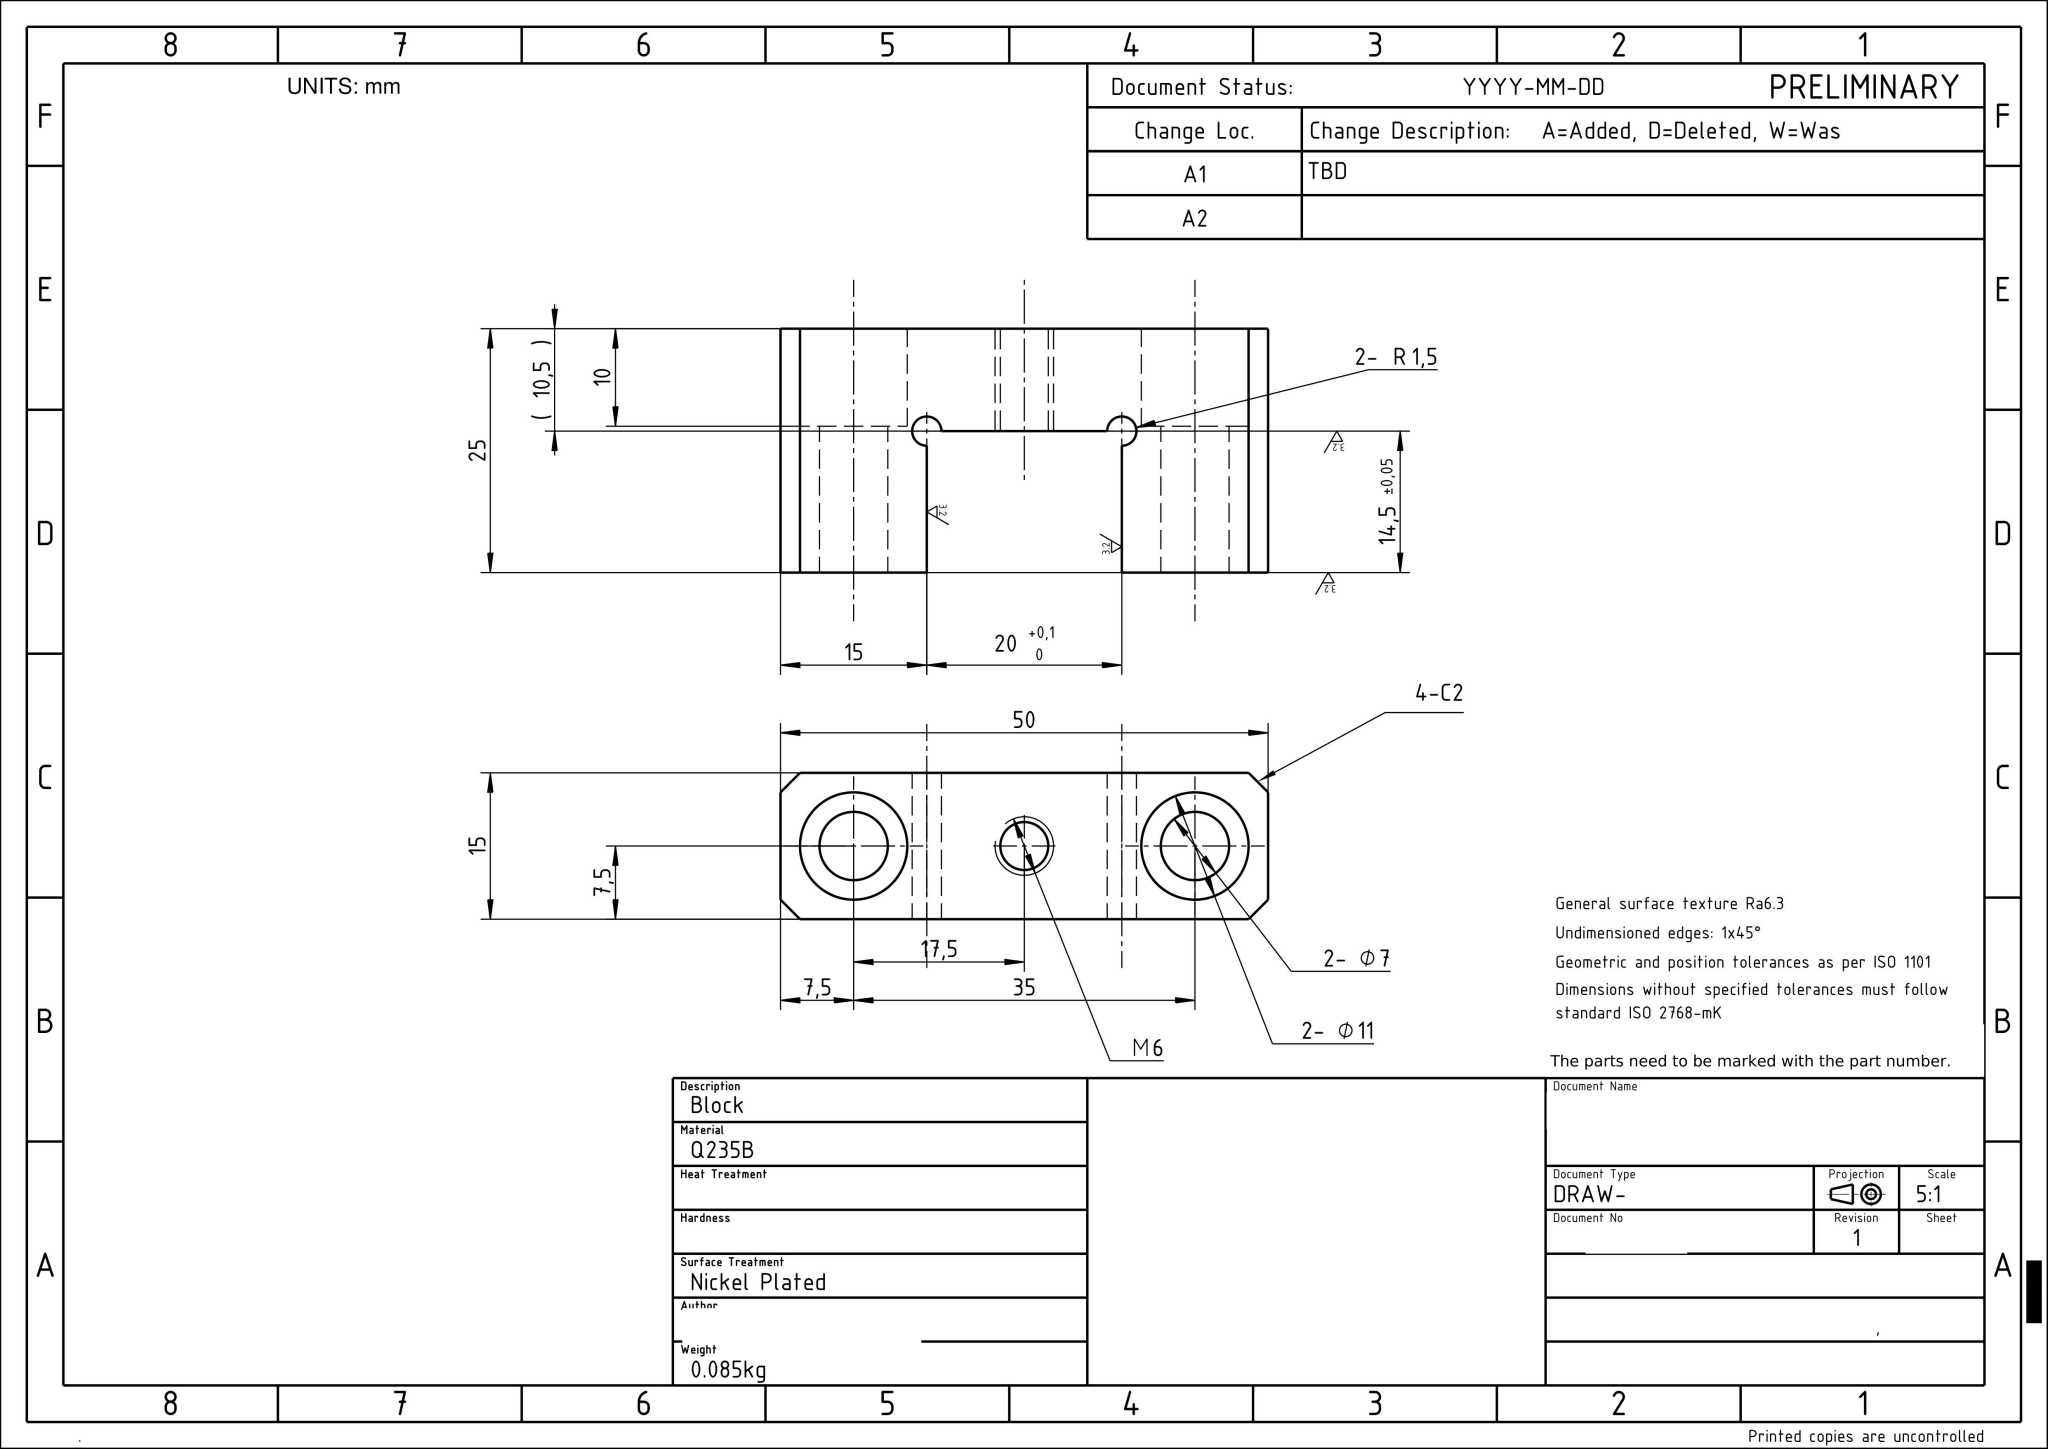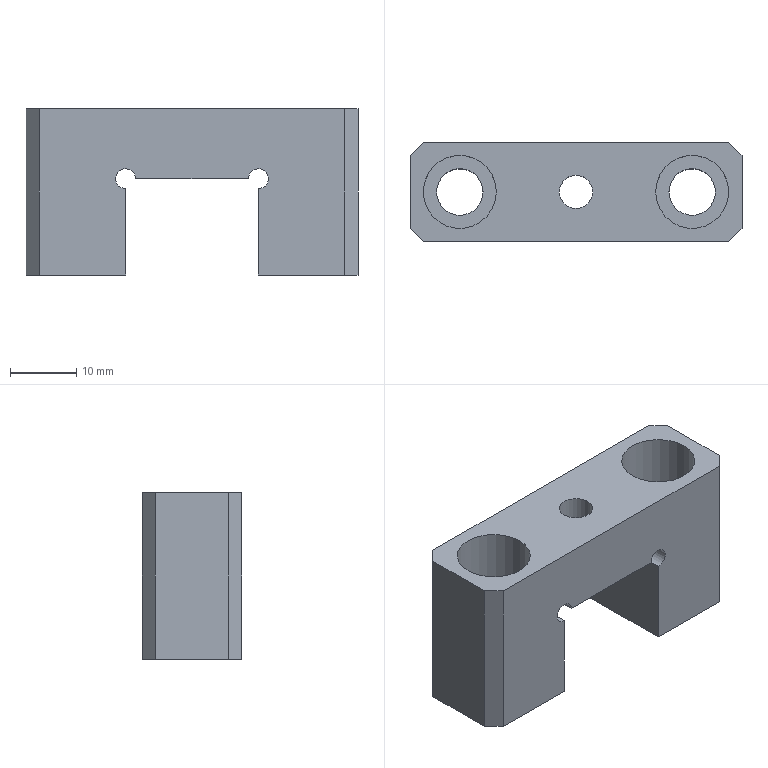Part | NX | mm | 1 solid | 23 faces | box 50 x 15 x 25 mm | volume 10780 mm3 | plane 16 | cylinder 7 | commonest cylinder face diameters 3 x2 7 x2 11 x2 5 x1
STEP:
#1=CARTESIAN_POINT('',(0.,0.,0.));
#2=DIRECTION('',(0.,0.,1.));
#3=DIRECTION('',(1.,0.,0.));
#4=AXIS2_PLACEMENT_3D('',#1,#2,#3);
#5=(LENGTH_UNIT()NAMED_UNIT(*)SI_UNIT(.MILLI.,.METRE.));
#6=UNCERTAINTY_MEASURE_WITH_UNIT(LENGTH_MEASURE(0.00002),#5,'','');
#7=(NAMED_UNIT(*)PLANE_ANGLE_UNIT()SI_UNIT($,.RADIAN.));
#8=PLANE_ANGLE_MEASURE_WITH_UNIT(PLANE_ANGLE_MEASURE(0.01745),#7);
#9=DIMENSIONAL_EXPONENTS(0.,0.,0.,0.,0.,0.,0.);
#10=(CONVERSION_BASED_UNIT('',#8)NAMED_UNIT(#9)PLANE_ANGLE_UNIT());
#11=(NAMED_UNIT(*)SI_UNIT($,.STERADIAN.)SOLID_ANGLE_UNIT());
#12=(GEOMETRIC_REPRESENTATION_CONTEXT(3)GLOBAL_UNCERTAINTY_ASSIGNED_CONTEXT((#6))GLOBAL_UNIT_ASSIGNED_CONTEXT((#5,#10,#11))REPRESENTATION_CONTEXT('',''));
#13=SHAPE_REPRESENTATION('',(#4),#12);
#14=CARTESIAN_POINT('',(21.,-0.,0.));
#15=VERTEX_POINT('',#14);
#16=CARTESIAN_POINT('',(17.5,-0.,0.));
#17=DIRECTION('',(0.,0.,1.));
#18=DIRECTION('',(1.,0.,0.));
#19=AXIS2_PLACEMENT_3D('',#16,#17,#18);
#20=CIRCLE('',#19,3.5);
#21=EDGE_CURVE('',#15,#15,#20,.T.);
#22=ORIENTED_EDGE('',*,*,#21,.T.);
#23=EDGE_LOOP('',(#22));
#24=FACE_BOUND('',#23,.T.);
#25=CARTESIAN_POINT('',(25.,-5.5,0.));
#26=VERTEX_POINT('',#25);
#27=CARTESIAN_POINT('',(25.,5.5,0.));
#28=VERTEX_POINT('',#27);
#29=CARTESIAN_POINT('',(25.,-7.5,0.));
#30=DIRECTION('',(-0.,1.,0.));
#31=VECTOR('',#30,1.);
#32=LINE('',#29,#31);
#33=EDGE_CURVE('',#26,#28,#32,.T.);
#34=ORIENTED_EDGE('',*,*,#33,.F.);
#35=CARTESIAN_POINT('',(23.,-7.5,0.));
#36=VERTEX_POINT('',#35);
#37=CARTESIAN_POINT('',(25.,-5.5,0.));
#38=DIRECTION('',(-0.7071,-0.7071,0.));
#39=VECTOR('',#38,1.);
#40=LINE('',#37,#39);
#41=EDGE_CURVE('',#26,#36,#40,.T.);
#42=ORIENTED_EDGE('',*,*,#41,.T.);
#43=CARTESIAN_POINT('',(10.,-7.5,0.));
#44=VERTEX_POINT('',#43);
#45=CARTESIAN_POINT('',(-25.,-7.5,0.));
#46=DIRECTION('',(1.,0.,0.));
#47=VECTOR('',#46,1.);
#48=LINE('',#45,#47);
#49=EDGE_CURVE('',#44,#36,#48,.T.);
#50=ORIENTED_EDGE('',*,*,#49,.F.);
#51=CARTESIAN_POINT('',(10.,7.5,0.));
#52=VERTEX_POINT('',#51);
#53=CARTESIAN_POINT('',(10.,17.5,0.));
#54=DIRECTION('',(0.,-1.,0.));
#55=VECTOR('',#54,1.);
#56=LINE('',#53,#55);
#57=EDGE_CURVE('',#52,#44,#56,.T.);
#58=ORIENTED_EDGE('',*,*,#57,.F.);
#59=CARTESIAN_POINT('',(23.,7.5,0.));
#60=VERTEX_POINT('',#59);
#61=CARTESIAN_POINT('',(25.,7.5,0.));
#62=DIRECTION('',(-1.,0.,0.));
#63=VECTOR('',#62,1.);
#64=LINE('',#61,#63);
#65=EDGE_CURVE('',#60,#52,#64,.T.);
#66=ORIENTED_EDGE('',*,*,#65,.F.);
#67=CARTESIAN_POINT('',(23.,7.5,0.));
#68=DIRECTION('',(0.7071,-0.7071,0.));
#69=VECTOR('',#68,1.);
#70=LINE('',#67,#69);
#71=EDGE_CURVE('',#60,#28,#70,.T.);
#72=ORIENTED_EDGE('',*,*,#71,.T.);
#73=EDGE_LOOP('',(#34,#42,#50,#58,#66,#72));
#74=FACE_BOUND('',#73,.T.);
#75=CARTESIAN_POINT('',(0.,0.,0.));
#76=DIRECTION('',(0.,0.,1.));
#77=DIRECTION('',(1.,0.,0.));
#78=AXIS2_PLACEMENT_3D('',#75,#76,#77);
#79=PLANE('',#78);
#80=ADVANCED_FACE('',(#24,#74),#79,.F.);
#81=CARTESIAN_POINT('',(-25.,5.5,25.));
#82=VERTEX_POINT('',#81);
#83=CARTESIAN_POINT('',(-25.,-5.5,25.));
#84=VERTEX_POINT('',#83);
#85=CARTESIAN_POINT('',(-25.,7.5,25.));
#86=DIRECTION('',(0.,-1.,0.));
#87=VECTOR('',#86,1.);
#88=LINE('',#85,#87);
#89=EDGE_CURVE('',#82,#84,#88,.T.);
#90=ORIENTED_EDGE('',*,*,#89,.F.);
#91=CARTESIAN_POINT('',(-25.,5.5,0.));
#92=VERTEX_POINT('',#91);
#93=CARTESIAN_POINT('',(-25.,5.5,25.));
#94=DIRECTION('',(0.,0.,-1.));
#95=VECTOR('',#94,1.);
#96=LINE('',#93,#95);
#97=EDGE_CURVE('',#82,#92,#96,.T.);
#98=ORIENTED_EDGE('',*,*,#97,.T.);
#99=CARTESIAN_POINT('',(-25.,-5.5,0.));
#100=VERTEX_POINT('',#99);
#101=CARTESIAN_POINT('',(-25.,7.5,0.));
#102=DIRECTION('',(0.,-1.,0.));
#103=VECTOR('',#102,1.);
#104=LINE('',#101,#103);
#105=EDGE_CURVE('',#92,#100,#104,.T.);
#106=ORIENTED_EDGE('',*,*,#105,.T.);
#107=CARTESIAN_POINT('',(-25.,-5.5,25.));
#108=DIRECTION('',(0.,0.,1.));
#109=VECTOR('',#108,1.);
#110=LINE('',#107,#109);
#111=EDGE_CURVE('',#100,#84,#110,.T.);
#112=ORIENTED_EDGE('',*,*,#111,.T.);
#113=EDGE_LOOP('',(#90,#98,#106,#112));
#114=FACE_OUTER_BOUND('',#113,.T.);
#115=CARTESIAN_POINT('',(-25.,7.5,25.));
#116=DIRECTION('',(1.,0.,0.));
#117=DIRECTION('',(-0.,1.,0.));
#118=AXIS2_PLACEMENT_3D('',#115,#116,#117);
#119=PLANE('',#118);
#120=ADVANCED_FACE('',(#114),#119,.F.);
#121=ORIENTED_EDGE('',*,*,#49,.T.);
#122=CARTESIAN_POINT('',(23.,-7.5,25.));
#123=VERTEX_POINT('',#122);
#124=CARTESIAN_POINT('',(23.,-7.5,25.));
#125=DIRECTION('',(0.,0.,1.));
#126=VECTOR('',#125,1.);
#127=LINE('',#124,#126);
#128=EDGE_CURVE('',#36,#123,#127,.T.);
#129=ORIENTED_EDGE('',*,*,#128,.T.);
#130=CARTESIAN_POINT('',(-23.,-7.5,25.));
#131=VERTEX_POINT('',#130);
#132=CARTESIAN_POINT('',(-25.,-7.5,25.));
#133=DIRECTION('',(1.,0.,0.));
#134=VECTOR('',#133,1.);
#135=LINE('',#132,#134);
#136=EDGE_CURVE('',#131,#123,#135,.T.);
#137=ORIENTED_EDGE('',*,*,#136,.F.);
#138=CARTESIAN_POINT('',(-23.,-7.5,0.));
#139=VERTEX_POINT('',#138);
#140=CARTESIAN_POINT('',(-23.,-7.5,25.));
#141=DIRECTION('',(0.,0.,-1.));
#142=VECTOR('',#141,1.);
#143=LINE('',#140,#142);
#144=EDGE_CURVE('',#131,#139,#143,.T.);
#145=ORIENTED_EDGE('',*,*,#144,.T.);
#146=CARTESIAN_POINT('',(-10.,-7.5,0.));
#147=VERTEX_POINT('',#146);
#148=CARTESIAN_POINT('',(-25.,-7.5,0.));
#149=DIRECTION('',(1.,0.,0.));
#150=VECTOR('',#149,1.);
#151=LINE('',#148,#150);
#152=EDGE_CURVE('',#139,#147,#151,.T.);
#153=ORIENTED_EDGE('',*,*,#152,.T.);
#154=CARTESIAN_POINT('',(-10.,-7.5,13.));
#155=VERTEX_POINT('',#154);
#156=CARTESIAN_POINT('',(-10.,-7.5,25.));
#157=DIRECTION('',(0.,0.,1.));
#158=VECTOR('',#157,1.);
#159=LINE('',#156,#158);
#160=EDGE_CURVE('',#147,#155,#159,.T.);
#161=ORIENTED_EDGE('',*,*,#160,.T.);
#162=CARTESIAN_POINT('',(-8.5,-7.5,14.5));
#163=VERTEX_POINT('',#162);
#164=CARTESIAN_POINT('',(-10.,-7.5,14.5));
#165=DIRECTION('',(0.,1.,0.));
#166=DIRECTION('',(0.,0.,1.));
#167=AXIS2_PLACEMENT_3D('',#164,#165,#166);
#168=CIRCLE('',#167,1.5);
#169=EDGE_CURVE('',#155,#163,#168,.T.);
#170=ORIENTED_EDGE('',*,*,#169,.T.);
#171=CARTESIAN_POINT('',(8.5,-7.5,14.5));
#172=VERTEX_POINT('',#171);
#173=CARTESIAN_POINT('',(-25.,-7.5,14.5));
#174=DIRECTION('',(1.,0.,0.));
#175=VECTOR('',#174,1.);
#176=LINE('',#173,#175);
#177=EDGE_CURVE('',#163,#172,#176,.T.);
#178=ORIENTED_EDGE('',*,*,#177,.T.);
#179=CARTESIAN_POINT('',(10.,-7.5,13.));
#180=VERTEX_POINT('',#179);
#181=CARTESIAN_POINT('',(10.,-7.5,14.5));
#182=DIRECTION('',(0.,1.,0.));
#183=DIRECTION('',(0.,0.,1.));
#184=AXIS2_PLACEMENT_3D('',#181,#182,#183);
#185=CIRCLE('',#184,1.5);
#186=EDGE_CURVE('',#172,#180,#185,.T.);
#187=ORIENTED_EDGE('',*,*,#186,.T.);
#188=CARTESIAN_POINT('',(10.,-7.5,25.));
#189=DIRECTION('',(0.,0.,-1.));
#190=VECTOR('',#189,1.);
#191=LINE('',#188,#190);
#192=EDGE_CURVE('',#180,#44,#191,.T.);
#193=ORIENTED_EDGE('',*,*,#192,.T.);
#194=EDGE_LOOP('',(#121,#129,#137,#145,#153,#161,#170,#178,#187,#193));
#195=FACE_OUTER_BOUND('',#194,.T.);
#196=CARTESIAN_POINT('',(-25.,-7.5,25.));
#197=DIRECTION('',(0.,1.,0.));
#198=DIRECTION('',(0.,0.,1.));
#199=AXIS2_PLACEMENT_3D('',#196,#197,#198);
#200=PLANE('',#199);
#201=ADVANCED_FACE('',(#195),#200,.F.);
#202=CARTESIAN_POINT('',(25.,-5.5,25.));
#203=VERTEX_POINT('',#202);
#204=CARTESIAN_POINT('',(25.,5.5,25.));
#205=VERTEX_POINT('',#204);
#206=CARTESIAN_POINT('',(25.,-7.5,25.));
#207=DIRECTION('',(-0.,1.,0.));
#208=VECTOR('',#207,1.);
#209=LINE('',#206,#208);
#210=EDGE_CURVE('',#203,#205,#209,.T.);
#211=ORIENTED_EDGE('',*,*,#210,.F.);
#212=CARTESIAN_POINT('',(25.,-5.5,25.));
#213=DIRECTION('',(0.,0.,-1.));
#214=VECTOR('',#213,1.);
#215=LINE('',#212,#214);
#216=EDGE_CURVE('',#203,#26,#215,.T.);
#217=ORIENTED_EDGE('',*,*,#216,.T.);
#218=ORIENTED_EDGE('',*,*,#33,.T.);
#219=CARTESIAN_POINT('',(25.,5.5,25.));
#220=DIRECTION('',(0.,0.,1.));
#221=VECTOR('',#220,1.);
#222=LINE('',#219,#221);
#223=EDGE_CURVE('',#28,#205,#222,.T.);
#224=ORIENTED_EDGE('',*,*,#223,.T.);
#225=EDGE_LOOP('',(#211,#217,#218,#224));
#226=FACE_OUTER_BOUND('',#225,.T.);
#227=CARTESIAN_POINT('',(25.,-7.5,25.));
#228=DIRECTION('',(-1.,-0.,0.));
#229=DIRECTION('',(0.,-1.,0.));
#230=AXIS2_PLACEMENT_3D('',#227,#228,#229);
#231=PLANE('',#230);
#232=ADVANCED_FACE('',(#226),#231,.F.);
#233=CARTESIAN_POINT('',(23.,7.5,25.));
#234=VERTEX_POINT('',#233);
#235=CARTESIAN_POINT('',(-23.,7.5,25.));
#236=VERTEX_POINT('',#235);
#237=CARTESIAN_POINT('',(25.,7.5,25.));
#238=DIRECTION('',(-1.,0.,0.));
#239=VECTOR('',#238,1.);
#240=LINE('',#237,#239);
#241=EDGE_CURVE('',#234,#236,#240,.T.);
#242=ORIENTED_EDGE('',*,*,#241,.F.);
#243=CARTESIAN_POINT('',(23.,7.5,25.));
#244=DIRECTION('',(0.,0.,-1.));
#245=VECTOR('',#244,1.);
#246=LINE('',#243,#245);
#247=EDGE_CURVE('',#234,#60,#246,.T.);
#248=ORIENTED_EDGE('',*,*,#247,.T.);
#249=ORIENTED_EDGE('',*,*,#65,.T.);
#250=CARTESIAN_POINT('',(10.,7.5,13.));
#251=VERTEX_POINT('',#250);
#252=CARTESIAN_POINT('',(10.,7.5,25.));
#253=DIRECTION('',(0.,0.,1.));
#254=VECTOR('',#253,1.);
#255=LINE('',#252,#254);
#256=EDGE_CURVE('',#52,#251,#255,.T.);
#257=ORIENTED_EDGE('',*,*,#256,.T.);
#258=CARTESIAN_POINT('',(8.5,7.5,14.5));
#259=VERTEX_POINT('',#258);
#260=CARTESIAN_POINT('',(10.,7.5,14.5));
#261=DIRECTION('',(0.,-1.,0.));
#262=DIRECTION('',(0.,0.,-1.));
#263=AXIS2_PLACEMENT_3D('',#260,#261,#262);
#264=CIRCLE('',#263,1.5);
#265=EDGE_CURVE('',#251,#259,#264,.T.);
#266=ORIENTED_EDGE('',*,*,#265,.T.);
#267=CARTESIAN_POINT('',(-8.5,7.5,14.5));
#268=VERTEX_POINT('',#267);
#269=CARTESIAN_POINT('',(25.,7.5,14.5));
#270=DIRECTION('',(-1.,0.,0.));
#271=VECTOR('',#270,1.);
#272=LINE('',#269,#271);
#273=EDGE_CURVE('',#259,#268,#272,.T.);
#274=ORIENTED_EDGE('',*,*,#273,.T.);
#275=CARTESIAN_POINT('',(-10.,7.5,13.));
#276=VERTEX_POINT('',#275);
#277=CARTESIAN_POINT('',(-10.,7.5,14.5));
#278=DIRECTION('',(0.,-1.,0.));
#279=DIRECTION('',(0.,0.,-1.));
#280=AXIS2_PLACEMENT_3D('',#277,#278,#279);
#281=CIRCLE('',#280,1.5);
#282=EDGE_CURVE('',#268,#276,#281,.T.);
#283=ORIENTED_EDGE('',*,*,#282,.T.);
#284=CARTESIAN_POINT('',(-10.,7.5,0.));
#285=VERTEX_POINT('',#284);
#286=CARTESIAN_POINT('',(-10.,7.5,25.));
#287=DIRECTION('',(0.,0.,-1.));
#288=VECTOR('',#287,1.);
#289=LINE('',#286,#288);
#290=EDGE_CURVE('',#276,#285,#289,.T.);
#291=ORIENTED_EDGE('',*,*,#290,.T.);
#292=CARTESIAN_POINT('',(-23.,7.5,0.));
#293=VERTEX_POINT('',#292);
#294=CARTESIAN_POINT('',(25.,7.5,0.));
#295=DIRECTION('',(-1.,0.,0.));
#296=VECTOR('',#295,1.);
#297=LINE('',#294,#296);
#298=EDGE_CURVE('',#285,#293,#297,.T.);
#299=ORIENTED_EDGE('',*,*,#298,.T.);
#300=CARTESIAN_POINT('',(-23.,7.5,25.));
#301=DIRECTION('',(0.,0.,1.));
#302=VECTOR('',#301,1.);
#303=LINE('',#300,#302);
#304=EDGE_CURVE('',#293,#236,#303,.T.);
#305=ORIENTED_EDGE('',*,*,#304,.T.);
#306=EDGE_LOOP('',(#242,#248,#249,#257,#266,#274,#283,#291,#299,#305));
#307=FACE_OUTER_BOUND('',#306,.T.);
#308=CARTESIAN_POINT('',(25.,7.5,25.));
#309=DIRECTION('',(0.,-1.,0.));
#310=DIRECTION('',(0.,0.,-1.));
#311=AXIS2_PLACEMENT_3D('',#308,#309,#310);
#312=PLANE('',#311);
#313=ADVANCED_FACE('',(#307),#312,.F.);
#314=CARTESIAN_POINT('',(12.,-0.,25.));
#315=VERTEX_POINT('',#314);
#316=CARTESIAN_POINT('',(17.5,-0.,25.));
#317=DIRECTION('',(0.,0.,-1.));
#318=DIRECTION('',(-1.,0.,0.));
#319=AXIS2_PLACEMENT_3D('',#316,#317,#318);
#320=CIRCLE('',#319,5.5);
#321=EDGE_CURVE('',#315,#315,#320,.T.);
#322=ORIENTED_EDGE('',*,*,#321,.T.);
#323=EDGE_LOOP('',(#322));
#324=FACE_BOUND('',#323,.T.);
#325=CARTESIAN_POINT('',(-23.,0.,25.));
#326=VERTEX_POINT('',#325);
#327=CARTESIAN_POINT('',(-17.5,0.,25.));
#328=DIRECTION('',(0.,0.,-1.));
#329=DIRECTION('',(-1.,0.,0.));
#330=AXIS2_PLACEMENT_3D('',#327,#328,#329);
#331=CIRCLE('',#330,5.5);
#332=EDGE_CURVE('',#326,#326,#331,.T.);
#333=ORIENTED_EDGE('',*,*,#332,.T.);
#334=EDGE_LOOP('',(#333));
#335=FACE_BOUND('',#334,.T.);
#336=CARTESIAN_POINT('',(-2.5,0.,25.));
#337=VERTEX_POINT('',#336);
#338=CARTESIAN_POINT('',(0.,0.,25.));
#339=DIRECTION('',(0.,0.,-1.));
#340=DIRECTION('',(-1.,0.,0.));
#341=AXIS2_PLACEMENT_3D('',#338,#339,#340);
#342=CIRCLE('',#341,2.5);
#343=EDGE_CURVE('',#337,#337,#342,.T.);
#344=ORIENTED_EDGE('',*,*,#343,.T.);
#345=EDGE_LOOP('',(#344));
#346=FACE_BOUND('',#345,.T.);
#347=ORIENTED_EDGE('',*,*,#136,.T.);
#348=CARTESIAN_POINT('',(15.25,-15.25,25.));
#349=DIRECTION('',(0.7071,0.7071,0.));
#350=VECTOR('',#349,1.);
#351=LINE('',#348,#350);
#352=EDGE_CURVE('',#123,#203,#351,.T.);
#353=ORIENTED_EDGE('',*,*,#352,.T.);
#354=ORIENTED_EDGE('',*,*,#210,.T.);
#355=CARTESIAN_POINT('',(15.25,15.25,25.));
#356=DIRECTION('',(-0.7071,0.7071,0.));
#357=VECTOR('',#356,1.);
#358=LINE('',#355,#357);
#359=EDGE_CURVE('',#205,#234,#358,.T.);
#360=ORIENTED_EDGE('',*,*,#359,.T.);
#361=ORIENTED_EDGE('',*,*,#241,.T.);
#362=CARTESIAN_POINT('',(-15.25,15.25,25.));
#363=DIRECTION('',(-0.7071,-0.7071,0.));
#364=VECTOR('',#363,1.);
#365=LINE('',#362,#364);
#366=EDGE_CURVE('',#236,#82,#365,.T.);
#367=ORIENTED_EDGE('',*,*,#366,.T.);
#368=ORIENTED_EDGE('',*,*,#89,.T.);
#369=CARTESIAN_POINT('',(-15.25,-15.25,25.));
#370=DIRECTION('',(0.7071,-0.7071,0.));
#371=VECTOR('',#370,1.);
#372=LINE('',#369,#371);
#373=EDGE_CURVE('',#84,#131,#372,.T.);
#374=ORIENTED_EDGE('',*,*,#373,.T.);
#375=EDGE_LOOP('',(#347,#353,#354,#360,#361,#367,#368,#374));
#376=FACE_BOUND('',#375,.T.);
#377=CARTESIAN_POINT('',(0.,0.,25.));
#378=DIRECTION('',(0.,0.,1.));
#379=DIRECTION('',(1.,0.,0.));
#380=AXIS2_PLACEMENT_3D('',#377,#378,#379);
#381=PLANE('',#380);
#382=ADVANCED_FACE('',(#324,#335,#346,#376),#381,.T.);
#383=CARTESIAN_POINT('',(-14.,0.,0.));
#384=VERTEX_POINT('',#383);
#385=CARTESIAN_POINT('',(-17.5,0.,0.));
#386=DIRECTION('',(0.,0.,1.));
#387=DIRECTION('',(1.,0.,0.));
#388=AXIS2_PLACEMENT_3D('',#385,#386,#387);
#389=CIRCLE('',#388,3.5);
#390=EDGE_CURVE('',#384,#384,#389,.T.);
#391=ORIENTED_EDGE('',*,*,#390,.T.);
#392=EDGE_LOOP('',(#391));
#393=FACE_BOUND('',#392,.T.);
#394=ORIENTED_EDGE('',*,*,#105,.F.);
#395=CARTESIAN_POINT('',(-25.,5.5,0.));
#396=DIRECTION('',(0.7071,0.7071,0.));
#397=VECTOR('',#396,1.);
#398=LINE('',#395,#397);
#399=EDGE_CURVE('',#92,#293,#398,.T.);
#400=ORIENTED_EDGE('',*,*,#399,.T.);
#401=ORIENTED_EDGE('',*,*,#298,.F.);
#402=CARTESIAN_POINT('',(-10.,17.5,0.));
#403=DIRECTION('',(0.,-1.,0.));
#404=VECTOR('',#403,1.);
#405=LINE('',#402,#404);
#406=EDGE_CURVE('',#285,#147,#405,.T.);
#407=ORIENTED_EDGE('',*,*,#406,.T.);
#408=ORIENTED_EDGE('',*,*,#152,.F.);
#409=CARTESIAN_POINT('',(-23.,-7.5,0.));
#410=DIRECTION('',(-0.7071,0.7071,0.));
#411=VECTOR('',#410,1.);
#412=LINE('',#409,#411);
#413=EDGE_CURVE('',#139,#100,#412,.T.);
#414=ORIENTED_EDGE('',*,*,#413,.T.);
#415=EDGE_LOOP('',(#394,#400,#401,#407,#408,#414));
#416=FACE_BOUND('',#415,.T.);
#417=CARTESIAN_POINT('',(0.,0.,0.));
#418=DIRECTION('',(0.,0.,1.));
#419=DIRECTION('',(1.,0.,0.));
#420=AXIS2_PLACEMENT_3D('',#417,#418,#419);
#421=PLANE('',#420);
#422=ADVANCED_FACE('',(#393,#416),#421,.F.);
#423=ORIENTED_EDGE('',*,*,#406,.F.);
#424=ORIENTED_EDGE('',*,*,#290,.F.);
#425=CARTESIAN_POINT('',(-10.,17.5,13.));
#426=DIRECTION('',(0.,1.,0.));
#427=VECTOR('',#426,1.);
#428=LINE('',#425,#427);
#429=EDGE_CURVE('',#155,#276,#428,.T.);
#430=ORIENTED_EDGE('',*,*,#429,.F.);
#431=ORIENTED_EDGE('',*,*,#160,.F.);
#432=EDGE_LOOP('',(#423,#424,#430,#431));
#433=FACE_OUTER_BOUND('',#432,.T.);
#434=CARTESIAN_POINT('',(-10.,17.5,13.));
#435=DIRECTION('',(-1.,0.,0.));
#436=DIRECTION('',(0.,0.,1.));
#437=AXIS2_PLACEMENT_3D('',#434,#435,#436);
#438=PLANE('',#437);
#439=ADVANCED_FACE('',(#433),#438,.F.);
#440=CARTESIAN_POINT('',(10.,17.5,13.));
#441=DIRECTION('',(0.,1.,0.));
#442=VECTOR('',#441,1.);
#443=LINE('',#440,#442);
#444=EDGE_CURVE('',#180,#251,#443,.T.);
#445=ORIENTED_EDGE('',*,*,#444,.T.);
#446=ORIENTED_EDGE('',*,*,#256,.F.);
#447=ORIENTED_EDGE('',*,*,#57,.T.);
#448=ORIENTED_EDGE('',*,*,#192,.F.);
#449=EDGE_LOOP('',(#445,#446,#447,#448));
#450=FACE_OUTER_BOUND('',#449,.T.);
#451=CARTESIAN_POINT('',(10.,17.5,0.));
#452=DIRECTION('',(1.,0.,0.));
#453=DIRECTION('',(0.,0.,-1.));
#454=AXIS2_PLACEMENT_3D('',#451,#452,#453);
#455=PLANE('',#454);
#456=ADVANCED_FACE('',(#450),#455,.F.);
#457=CARTESIAN_POINT('',(8.5,17.5,14.5));
#458=DIRECTION('',(0.,1.,0.));
#459=VECTOR('',#458,1.);
#460=LINE('',#457,#459);
#461=EDGE_CURVE('',#172,#259,#460,.T.);
#462=ORIENTED_EDGE('',*,*,#461,.T.);
#463=ORIENTED_EDGE('',*,*,#265,.F.);
#464=ORIENTED_EDGE('',*,*,#444,.F.);
#465=ORIENTED_EDGE('',*,*,#186,.F.);
#466=EDGE_LOOP('',(#462,#463,#464,#465));
#467=FACE_OUTER_BOUND('',#466,.T.);
#468=CARTESIAN_POINT('',(10.,17.5,14.5));
#469=DIRECTION('',(0.,-1.,0.));
#470=DIRECTION('',(0.,0.,-1.));
#471=AXIS2_PLACEMENT_3D('',#468,#469,#470);
#472=CYLINDRICAL_SURFACE('',#471,1.5);
#473=ADVANCED_FACE('',(#467),#472,.F.);
#474=CARTESIAN_POINT('',(2.5,0.,14.5));
#475=VERTEX_POINT('',#474);
#476=CARTESIAN_POINT('',(0.,0.,14.5));
#477=DIRECTION('',(0.,0.,1.));
#478=DIRECTION('',(1.,0.,0.));
#479=AXIS2_PLACEMENT_3D('',#476,#477,#478);
#480=CIRCLE('',#479,2.5);
#481=EDGE_CURVE('',#475,#475,#480,.T.);
#482=ORIENTED_EDGE('',*,*,#481,.T.);
#483=EDGE_LOOP('',(#482));
#484=FACE_BOUND('',#483,.T.);
#485=CARTESIAN_POINT('',(-8.5,17.5,14.5));
#486=DIRECTION('',(0.,1.,0.));
#487=VECTOR('',#486,1.);
#488=LINE('',#485,#487);
#489=EDGE_CURVE('',#163,#268,#488,.T.);
#490=ORIENTED_EDGE('',*,*,#489,.T.);
#491=ORIENTED_EDGE('',*,*,#273,.F.);
#492=ORIENTED_EDGE('',*,*,#461,.F.);
#493=ORIENTED_EDGE('',*,*,#177,.F.);
#494=EDGE_LOOP('',(#490,#491,#492,#493));
#495=FACE_BOUND('',#494,.T.);
#496=CARTESIAN_POINT('',(8.5,17.5,14.5));
#497=DIRECTION('',(0.,0.,1.));
#498=DIRECTION('',(1.,0.,0.));
#499=AXIS2_PLACEMENT_3D('',#496,#497,#498);
#500=PLANE('',#499);
#501=ADVANCED_FACE('',(#484,#495),#500,.F.);
#502=ORIENTED_EDGE('',*,*,#429,.T.);
#503=ORIENTED_EDGE('',*,*,#282,.F.);
#504=ORIENTED_EDGE('',*,*,#489,.F.);
#505=ORIENTED_EDGE('',*,*,#169,.F.);
#506=EDGE_LOOP('',(#502,#503,#504,#505));
#507=FACE_OUTER_BOUND('',#506,.T.);
#508=CARTESIAN_POINT('',(-10.,17.5,14.5));
#509=DIRECTION('',(0.,-1.,0.));
#510=DIRECTION('',(0.,0.,-1.));
#511=AXIS2_PLACEMENT_3D('',#508,#509,#510);
#512=CYLINDRICAL_SURFACE('',#511,1.5);
#513=ADVANCED_FACE('',(#507),#512,.F.);
#514=ORIENTED_EDGE('',*,*,#343,.F.);
#515=EDGE_LOOP('',(#514));
#516=FACE_BOUND('',#515,.T.);
#517=ORIENTED_EDGE('',*,*,#481,.F.);
#518=EDGE_LOOP('',(#517));
#519=FACE_BOUND('',#518,.T.);
#520=CARTESIAN_POINT('',(0.,0.,25.));
#521=DIRECTION('',(0.,0.,-1.));
#522=DIRECTION('',(-1.,0.,0.));
#523=AXIS2_PLACEMENT_3D('',#520,#521,#522);
#524=CYLINDRICAL_SURFACE('',#523,2.5);
#525=ADVANCED_FACE('',(#516,#519),#524,.F.);
#526=CARTESIAN_POINT('',(-21.,0.,15.));
#527=VERTEX_POINT('',#526);
#528=CARTESIAN_POINT('',(-17.5,0.,15.));
#529=DIRECTION('',(0.,0.,1.));
#530=DIRECTION('',(-1.,0.,0.));
#531=AXIS2_PLACEMENT_3D('',#528,#529,#530);
#532=CIRCLE('',#531,3.5);
#533=EDGE_CURVE('',#527,#527,#532,.T.);
#534=ORIENTED_EDGE('',*,*,#533,.T.);
#535=EDGE_LOOP('',(#534));
#536=FACE_BOUND('',#535,.T.);
#537=ORIENTED_EDGE('',*,*,#390,.F.);
#538=EDGE_LOOP('',(#537));
#539=FACE_BOUND('',#538,.T.);
#540=CARTESIAN_POINT('',(-17.5,0.,-14.092));
#541=DIRECTION('',(0.,0.,-1.));
#542=DIRECTION('',(-1.,0.,0.));
#543=AXIS2_PLACEMENT_3D('',#540,#541,#542);
#544=CYLINDRICAL_SURFACE('',#543,3.5);
#545=ADVANCED_FACE('',(#536,#539),#544,.F.);
#546=ORIENTED_EDGE('',*,*,#533,.F.);
#547=EDGE_LOOP('',(#546));
#548=FACE_BOUND('',#547,.T.);
#549=CARTESIAN_POINT('',(-23.,0.,15.));
#550=VERTEX_POINT('',#549);
#551=CARTESIAN_POINT('',(-17.5,0.,15.));
#552=DIRECTION('',(0.,0.,1.));
#553=DIRECTION('',(-1.,0.,0.));
#554=AXIS2_PLACEMENT_3D('',#551,#552,#553);
#555=CIRCLE('',#554,5.5);
#556=EDGE_CURVE('',#550,#550,#555,.T.);
#557=ORIENTED_EDGE('',*,*,#556,.T.);
#558=EDGE_LOOP('',(#557));
#559=FACE_BOUND('',#558,.T.);
#560=CARTESIAN_POINT('',(-17.5,0.,15.));
#561=DIRECTION('',(0.,0.,-1.));
#562=DIRECTION('',(-1.,0.,0.));
#563=AXIS2_PLACEMENT_3D('',#560,#561,#562);
#564=PLANE('',#563);
#565=ADVANCED_FACE('',(#548,#559),#564,.F.);
#566=ORIENTED_EDGE('',*,*,#556,.F.);
#567=EDGE_LOOP('',(#566));
#568=FACE_BOUND('',#567,.T.);
#569=ORIENTED_EDGE('',*,*,#332,.F.);
#570=EDGE_LOOP('',(#569));
#571=FACE_BOUND('',#570,.T.);
#572=CARTESIAN_POINT('',(-17.5,0.,25.));
#573=DIRECTION('',(0.,0.,-1.));
#574=DIRECTION('',(-1.,0.,0.));
#575=AXIS2_PLACEMENT_3D('',#572,#573,#574);
#576=CYLINDRICAL_SURFACE('',#575,5.5);
#577=ADVANCED_FACE('',(#568,#571),#576,.F.);
#578=CARTESIAN_POINT('',(14.,-0.,15.));
#579=VERTEX_POINT('',#578);
#580=CARTESIAN_POINT('',(17.5,-0.,15.));
#581=DIRECTION('',(0.,0.,1.));
#582=DIRECTION('',(-1.,0.,0.));
#583=AXIS2_PLACEMENT_3D('',#580,#581,#582);
#584=CIRCLE('',#583,3.5);
#585=EDGE_CURVE('',#579,#579,#584,.T.);
#586=ORIENTED_EDGE('',*,*,#585,.T.);
#587=EDGE_LOOP('',(#586));
#588=FACE_BOUND('',#587,.T.);
#589=ORIENTED_EDGE('',*,*,#21,.F.);
#590=EDGE_LOOP('',(#589));
#591=FACE_BOUND('',#590,.T.);
#592=CARTESIAN_POINT('',(17.5,-0.,-14.092));
#593=DIRECTION('',(0.,0.,-1.));
#594=DIRECTION('',(-1.,0.,0.));
#595=AXIS2_PLACEMENT_3D('',#592,#593,#594);
#596=CYLINDRICAL_SURFACE('',#595,3.5);
#597=ADVANCED_FACE('',(#588,#591),#596,.F.);
#598=ORIENTED_EDGE('',*,*,#585,.F.);
#599=EDGE_LOOP('',(#598));
#600=FACE_BOUND('',#599,.T.);
#601=CARTESIAN_POINT('',(12.,-0.,15.));
#602=VERTEX_POINT('',#601);
#603=CARTESIAN_POINT('',(17.5,-0.,15.));
#604=DIRECTION('',(0.,0.,1.));
#605=DIRECTION('',(-1.,0.,0.));
#606=AXIS2_PLACEMENT_3D('',#603,#604,#605);
#607=CIRCLE('',#606,5.5);
#608=EDGE_CURVE('',#602,#602,#607,.T.);
#609=ORIENTED_EDGE('',*,*,#608,.T.);
#610=EDGE_LOOP('',(#609));
#611=FACE_BOUND('',#610,.T.);
#612=CARTESIAN_POINT('',(17.5,-0.,15.));
#613=DIRECTION('',(0.,0.,-1.));
#614=DIRECTION('',(-1.,0.,0.));
#615=AXIS2_PLACEMENT_3D('',#612,#613,#614);
#616=PLANE('',#615);
#617=ADVANCED_FACE('',(#600,#611),#616,.F.);
#618=ORIENTED_EDGE('',*,*,#608,.F.);
#619=EDGE_LOOP('',(#618));
#620=FACE_BOUND('',#619,.T.);
#621=ORIENTED_EDGE('',*,*,#321,.F.);
#622=EDGE_LOOP('',(#621));
#623=FACE_BOUND('',#622,.T.);
#624=CARTESIAN_POINT('',(17.5,-0.,25.));
#625=DIRECTION('',(0.,0.,-1.));
#626=DIRECTION('',(-1.,0.,0.));
#627=AXIS2_PLACEMENT_3D('',#624,#625,#626);
#628=CYLINDRICAL_SURFACE('',#627,5.5);
#629=ADVANCED_FACE('',(#620,#623),#628,.F.);
#630=ORIENTED_EDGE('',*,*,#352,.F.);
#631=ORIENTED_EDGE('',*,*,#128,.F.);
#632=ORIENTED_EDGE('',*,*,#41,.F.);
#633=ORIENTED_EDGE('',*,*,#216,.F.);
#634=EDGE_LOOP('',(#630,#631,#632,#633));
#635=FACE_OUTER_BOUND('',#634,.T.);
#636=CARTESIAN_POINT('',(25.,-5.5,25.));
#637=DIRECTION('',(-0.7071,0.7071,0.));
#638=DIRECTION('',(0.,0.,-1.));
#639=AXIS2_PLACEMENT_3D('',#636,#637,#638);
#640=PLANE('',#639);
#641=ADVANCED_FACE('',(#635),#640,.F.);
#642=ORIENTED_EDGE('',*,*,#359,.F.);
#643=ORIENTED_EDGE('',*,*,#223,.F.);
#644=ORIENTED_EDGE('',*,*,#71,.F.);
#645=ORIENTED_EDGE('',*,*,#247,.F.);
#646=EDGE_LOOP('',(#642,#643,#644,#645));
#647=FACE_OUTER_BOUND('',#646,.T.);
#648=CARTESIAN_POINT('',(23.,7.5,25.));
#649=DIRECTION('',(-0.7071,-0.7071,0.));
#650=DIRECTION('',(0.,0.,-1.));
#651=AXIS2_PLACEMENT_3D('',#648,#649,#650);
#652=PLANE('',#651);
#653=ADVANCED_FACE('',(#647),#652,.F.);
#654=ORIENTED_EDGE('',*,*,#366,.F.);
#655=ORIENTED_EDGE('',*,*,#304,.F.);
#656=ORIENTED_EDGE('',*,*,#399,.F.);
#657=ORIENTED_EDGE('',*,*,#97,.F.);
#658=EDGE_LOOP('',(#654,#655,#656,#657));
#659=FACE_OUTER_BOUND('',#658,.T.);
#660=CARTESIAN_POINT('',(-25.,5.5,25.));
#661=DIRECTION('',(0.7071,-0.7071,0.));
#662=DIRECTION('',(0.,0.,-1.));
#663=AXIS2_PLACEMENT_3D('',#660,#661,#662);
#664=PLANE('',#663);
#665=ADVANCED_FACE('',(#659),#664,.F.);
#666=ORIENTED_EDGE('',*,*,#373,.F.);
#667=ORIENTED_EDGE('',*,*,#111,.F.);
#668=ORIENTED_EDGE('',*,*,#413,.F.);
#669=ORIENTED_EDGE('',*,*,#144,.F.);
#670=EDGE_LOOP('',(#666,#667,#668,#669));
#671=FACE_OUTER_BOUND('',#670,.T.);
#672=CARTESIAN_POINT('',(-23.,-7.5,25.));
#673=DIRECTION('',(0.7071,0.7071,0.));
#674=DIRECTION('',(0.,0.,-1.));
#675=AXIS2_PLACEMENT_3D('',#672,#673,#674);
#676=PLANE('',#675);
#677=ADVANCED_FACE('',(#671),#676,.F.);
#678=CLOSED_SHELL('',(#80,#120,#201,#232,#313,#382,#422,#439,#456,#473,#501,#513,#525,#545,#565,#577,#597,#617,#629,#641,#653,#665,#677));
#679=MANIFOLD_SOLID_BREP('',#678);
#680=ADVANCED_BREP_SHAPE_REPRESENTATION('',(#679),#12);
#681=SHAPE_REPRESENTATION_RELATIONSHIP('','',#13,#680);
#682=PRESENTATION_LAYER_ASSIGNMENT('','',(#679));
#683=COLOUR_RGB('',0.4,0.8,1.);
#684=FILL_AREA_STYLE_COLOUR('',#683);
#685=FILL_AREA_STYLE('',(#684));
#686=SURFACE_STYLE_FILL_AREA(#685);
#687=SURFACE_SIDE_STYLE('',(#686));
#688=SURFACE_STYLE_USAGE(.BOTH.,#687);
#689=PRESENTATION_STYLE_ASSIGNMENT((#688));
#690=STYLED_ITEM('',(#689),#679);
#691=MECHANICAL_DESIGN_GEOMETRIC_PRESENTATION_REPRESENTATION('',(#690),#12);